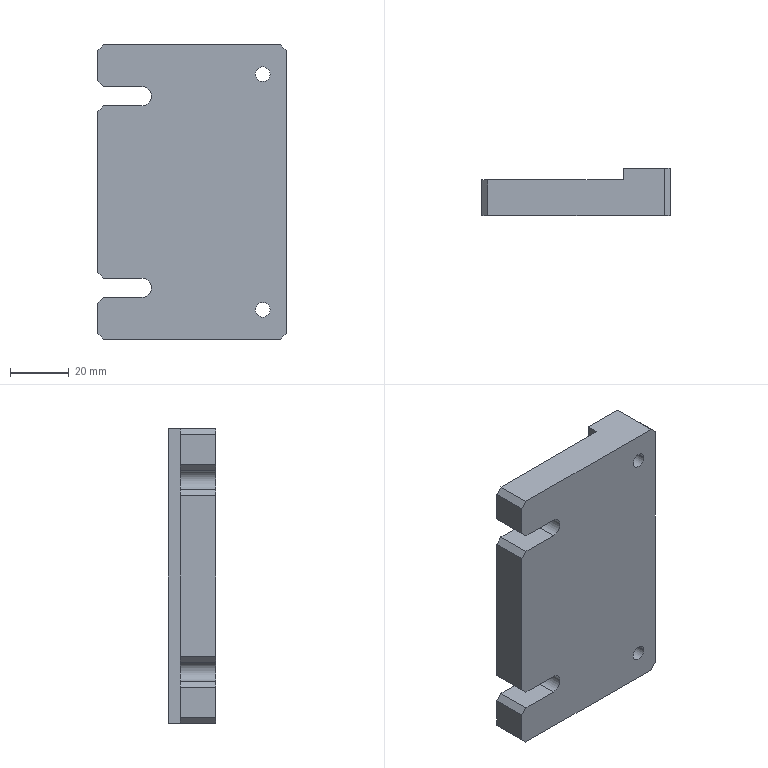Component | SolidWorks | 140507-L01M08U05-2-P03(B)-2 | 1 solid | 28 faces | box 64 x 16 x 100 mm | volume 79625 mm3 | plane 22 | cylinder 6 | commonest cylinder face diameters 5 x4 6.5 x2
build123d program:
from build123d import *

# Parameters (mm, degrees)
SKETCH1_W           = 100
SKETCH1_H           = 64
BOSS_EXTRUDE1_DEPTH = 16
CHAMFER1_SIZE       = 2
M6_TAPPED_HOLE1_D   = 5
CUT_EXTRUDE1_DEPTH  = 62.482
CHAMFER2_SIZE       = 2
SKETCH7_W           = 100
SKETCH7_H           = 48
CUT_EXTRUDE2_DEPTH  = 4


with BuildPart() as part:
    # Sketch1 → Boss-Extrude1 (new body)
    with BuildSketch(Plane(origin=(0, 0, 0), x_dir=(1, 0, 0), z_dir=(0, 1, 0))):
        Rectangle(SKETCH1_W, SKETCH1_H)
    extrude(amount=BOSS_EXTRUDE1_DEPTH)

    # Chamfer1
    chamfer1_edges = [part.edges().sort_by_distance(p)[0] for p in [
        (50, 8, 32),
        (-50, 8, 32),
        (-50, 8, -32),
        (50, 8, -32),
    ]]
    chamfer(chamfer1_edges, length=CHAMFER1_SIZE)

    # M6 Tapped Hole1 (through all)
    with Locations(Plane(origin=(0, 16, 0), x_dir=(1, 0, 0), z_dir=(0, 1, 0))):
        with Locations((-40, 24), (40, 24)):
            Hole(M6_TAPPED_HOLE1_D / 2)

    # Sketch6 → Cut-Extrude1 (cut, through all)
    with BuildSketch(Plane(origin=(0, 16, 0), x_dir=(1, 0, 0), z_dir=(0, 1, 0))):
        with BuildLine():
            Line((-35.75, -32), (-35.75, -17))
            ThreePointArc((-35.75, -17), (-32.5, -13.75), (-29.25, -17))
            Line((-29.25, -17), (-29.25, -32))
            ThreePointArc((-29.25, -32), (-32.5, -35.25), (-35.75, -32))
        make_face()
        with BuildLine():
            Line((35.75, -32), (35.75, -17))
            ThreePointArc((35.75, -17), (32.5, -13.75), (29.25, -17))
            Line((29.25, -17), (29.25, -32))
            ThreePointArc((29.25, -32), (32.5, -35.25), (35.75, -32))
        make_face()
    extrude(amount=-CUT_EXTRUDE1_DEPTH, mode=Mode.SUBTRACT)

    # Chamfer2
    chamfer2_edges = [part.edges().sort_by_distance(p)[0] for p in [
        (-29.25, 8, 32),
        (-35.75, 8, 32),
        (35.75, 8, 32),
        (29.25, 8, 32),
    ]]
    chamfer(chamfer2_edges, length=CHAMFER2_SIZE)

    # Sketch7 → Cut-Extrude2 (cut)
    with BuildSketch(Plane(origin=(0, 16, 0), x_dir=(1, 0, 0), z_dir=(0, 1, 0))):
        with Locations((0, -8)):
            Rectangle(SKETCH7_W, SKETCH7_H)
    extrude(amount=-CUT_EXTRUDE2_DEPTH, mode=Mode.SUBTRACT)


solid = part.part

# Placed as in the assembly
solid = solid.moved(Location((-58.945, -17.656, -21.398), (0, -90, 0)))
STEP:
#1=COLOUR_RGB('',0.7922,0.8196,0.9333);
#2=FILL_AREA_STYLE_COLOUR('',#1);
#3=FILL_AREA_STYLE('',(#2));
#4=SURFACE_STYLE_FILL_AREA(#3);
#5=SURFACE_SIDE_STYLE('',(#4));
#6=SURFACE_STYLE_USAGE(.BOTH.,#5);
#7=PRESENTATION_STYLE_ASSIGNMENT((#6));
#8=CARTESIAN_POINT('',(-1.277,-0.6951,-2.417));
#9=VERTEX_POINT('',#8);
#10=CARTESIAN_POINT('',(-1.474,-0.6951,-2.417));
#11=VERTEX_POINT('',#10);
#12=CARTESIAN_POINT('',(-1.376,-0.6951,-2.417));
#13=DIRECTION('',(0.,1.,0.));
#14=DIRECTION('',(-1.,0.,0.));
#15=AXIS2_PLACEMENT_3D('',#12,#13,#14);
#16=CIRCLE('',#15,0.09843);
#17=EDGE_CURVE('',#9,#11,#16,.T.);
#18=ORIENTED_EDGE('',*,*,#17,.F.);
#19=CARTESIAN_POINT('',(-1.277,-0.0652,-2.417));
#20=VERTEX_POINT('',#19);
#21=CARTESIAN_POINT('',(-1.277,-0.0652,-2.417));
#22=DIRECTION('',(0.,1.,0.));
#23=VECTOR('',#22,39.37);
#24=LINE('',#21,#23);
#25=EDGE_CURVE('',#9,#20,#24,.T.);
#26=ORIENTED_EDGE('',*,*,#25,.T.);
#27=CARTESIAN_POINT('',(-1.474,-0.0652,-2.417));
#28=VERTEX_POINT('',#27);
#29=CARTESIAN_POINT('',(-1.376,-0.0652,-2.417));
#30=DIRECTION('',(0.,1.,0.));
#31=DIRECTION('',(-1.,0.,0.));
#32=AXIS2_PLACEMENT_3D('',#29,#30,#31);
#33=CIRCLE('',#32,0.09843);
#34=EDGE_CURVE('',#20,#28,#33,.T.);
#35=ORIENTED_EDGE('',*,*,#34,.T.);
#36=CARTESIAN_POINT('',(-1.474,-0.0652,-2.417));
#37=DIRECTION('',(0.,1.,0.));
#38=VECTOR('',#37,39.37);
#39=LINE('',#36,#38);
#40=EDGE_CURVE('',#11,#28,#39,.T.);
#41=ORIENTED_EDGE('',*,*,#40,.F.);
#42=EDGE_LOOP('',(#18,#26,#35,#41));
#43=FACE_OUTER_BOUND('',#42,.T.);
#44=CARTESIAN_POINT('',(-1.376,-0.0652,-2.417));
#45=DIRECTION('',(0.,1.,0.));
#46=DIRECTION('',(-1.,0.,0.));
#47=AXIS2_PLACEMENT_3D('',#44,#45,#46);
#48=CYLINDRICAL_SURFACE('',#47,0.09843);
#49=ADVANCED_FACE('',(#43),#48,.F.);
#50=CARTESIAN_POINT('',(-1.277,-0.6951,0.7324));
#51=VERTEX_POINT('',#50);
#52=CARTESIAN_POINT('',(-1.474,-0.6951,0.7324));
#53=VERTEX_POINT('',#52);
#54=CARTESIAN_POINT('',(-1.376,-0.6951,0.7324));
#55=DIRECTION('',(0.,1.,0.));
#56=DIRECTION('',(-1.,0.,0.));
#57=AXIS2_PLACEMENT_3D('',#54,#55,#56);
#58=CIRCLE('',#57,0.09843);
#59=EDGE_CURVE('',#51,#53,#58,.T.);
#60=ORIENTED_EDGE('',*,*,#59,.F.);
#61=CARTESIAN_POINT('',(-1.277,-0.0652,0.7324));
#62=VERTEX_POINT('',#61);
#63=CARTESIAN_POINT('',(-1.277,-0.0652,0.7324));
#64=DIRECTION('',(0.,1.,0.));
#65=VECTOR('',#64,39.37);
#66=LINE('',#63,#65);
#67=EDGE_CURVE('',#51,#62,#66,.T.);
#68=ORIENTED_EDGE('',*,*,#67,.T.);
#69=CARTESIAN_POINT('',(-1.474,-0.0652,0.7324));
#70=VERTEX_POINT('',#69);
#71=CARTESIAN_POINT('',(-1.376,-0.0652,0.7324));
#72=DIRECTION('',(0.,1.,0.));
#73=DIRECTION('',(-1.,0.,0.));
#74=AXIS2_PLACEMENT_3D('',#71,#72,#73);
#75=CIRCLE('',#74,0.09843);
#76=EDGE_CURVE('',#62,#70,#75,.T.);
#77=ORIENTED_EDGE('',*,*,#76,.T.);
#78=CARTESIAN_POINT('',(-1.474,-0.0652,0.7324));
#79=DIRECTION('',(0.,1.,0.));
#80=VECTOR('',#79,39.37);
#81=LINE('',#78,#80);
#82=EDGE_CURVE('',#53,#70,#81,.T.);
#83=ORIENTED_EDGE('',*,*,#82,.F.);
#84=EDGE_LOOP('',(#60,#68,#77,#83));
#85=FACE_OUTER_BOUND('',#84,.T.);
#86=CARTESIAN_POINT('',(-1.376,-0.0652,0.7324));
#87=DIRECTION('',(0.,1.,0.));
#88=DIRECTION('',(-1.,0.,0.));
#89=AXIS2_PLACEMENT_3D('',#86,#87,#88);
#90=CYLINDRICAL_SURFACE('',#89,0.09843);
#91=ADVANCED_FACE('',(#85),#90,.F.);
#92=CARTESIAN_POINT('',(-3.581,-0.2227,-1.915));
#93=VERTEX_POINT('',#92);
#94=CARTESIAN_POINT('',(-3.581,-0.2227,0.2304));
#95=VERTEX_POINT('',#94);
#96=CARTESIAN_POINT('',(-3.581,-0.2227,-2.811));
#97=DIRECTION('',(-0.,-0.,1.));
#98=VECTOR('',#97,39.37);
#99=LINE('',#96,#98);
#100=EDGE_CURVE('',#93,#95,#99,.T.);
#101=ORIENTED_EDGE('',*,*,#100,.F.);
#102=CARTESIAN_POINT('',(-3.581,-0.6951,-1.915));
#103=VERTEX_POINT('',#102);
#104=CARTESIAN_POINT('',(-3.581,-0.0652,-1.915));
#105=DIRECTION('',(-0.,-1.,-0.));
#106=VECTOR('',#105,39.37);
#107=LINE('',#104,#106);
#108=EDGE_CURVE('',#93,#103,#107,.T.);
#109=ORIENTED_EDGE('',*,*,#108,.T.);
#110=CARTESIAN_POINT('',(-3.581,-0.6951,0.2304));
#111=VERTEX_POINT('',#110);
#112=CARTESIAN_POINT('',(-3.581,-0.6951,-2.811));
#113=DIRECTION('',(-0.,-0.,1.));
#114=VECTOR('',#113,39.37);
#115=LINE('',#112,#114);
#116=EDGE_CURVE('',#103,#111,#115,.T.);
#117=ORIENTED_EDGE('',*,*,#116,.T.);
#118=CARTESIAN_POINT('',(-3.581,-0.0652,0.2304));
#119=DIRECTION('',(0.,1.,0.));
#120=VECTOR('',#119,39.37);
#121=LINE('',#118,#120);
#122=EDGE_CURVE('',#111,#95,#121,.T.);
#123=ORIENTED_EDGE('',*,*,#122,.T.);
#124=EDGE_LOOP('',(#101,#109,#117,#123));
#125=FACE_OUTER_BOUND('',#124,.T.);
#126=CARTESIAN_POINT('',(-3.581,-0.0652,-2.811));
#127=DIRECTION('',(1.,-0.,0.));
#128=DIRECTION('',(0.,0.,-1.));
#129=AXIS2_PLACEMENT_3D('',#126,#127,#128);
#130=PLANE('',#129);
#131=ADVANCED_FACE('',(#125),#130,.F.);
#132=CARTESIAN_POINT('',(-3.581,-0.2227,-2.732));
#133=VERTEX_POINT('',#132);
#134=CARTESIAN_POINT('',(-3.581,-0.2227,-2.329));
#135=VERTEX_POINT('',#134);
#136=CARTESIAN_POINT('',(-3.581,-0.2227,-2.811));
#137=DIRECTION('',(-0.,-0.,1.));
#138=VECTOR('',#137,39.37);
#139=LINE('',#136,#138);
#140=EDGE_CURVE('',#133,#135,#139,.T.);
#141=ORIENTED_EDGE('',*,*,#140,.F.);
#142=CARTESIAN_POINT('',(-3.581,-0.6951,-2.732));
#143=VERTEX_POINT('',#142);
#144=CARTESIAN_POINT('',(-3.581,-0.0652,-2.732));
#145=DIRECTION('',(-0.,-1.,-0.));
#146=VECTOR('',#145,39.37);
#147=LINE('',#144,#146);
#148=EDGE_CURVE('',#133,#143,#147,.T.);
#149=ORIENTED_EDGE('',*,*,#148,.T.);
#150=CARTESIAN_POINT('',(-3.581,-0.6951,-2.329));
#151=VERTEX_POINT('',#150);
#152=CARTESIAN_POINT('',(-3.581,-0.6951,-2.811));
#153=DIRECTION('',(-0.,-0.,1.));
#154=VECTOR('',#153,39.37);
#155=LINE('',#152,#154);
#156=EDGE_CURVE('',#143,#151,#155,.T.);
#157=ORIENTED_EDGE('',*,*,#156,.T.);
#158=CARTESIAN_POINT('',(-3.581,-0.0652,-2.329));
#159=DIRECTION('',(0.,1.,0.));
#160=VECTOR('',#159,39.37);
#161=LINE('',#158,#160);
#162=EDGE_CURVE('',#151,#135,#161,.T.);
#163=ORIENTED_EDGE('',*,*,#162,.T.);
#164=EDGE_LOOP('',(#141,#149,#157,#163));
#165=FACE_OUTER_BOUND('',#164,.T.);
#166=CARTESIAN_POINT('',(-3.581,-0.0652,-2.811));
#167=DIRECTION('',(1.,-0.,0.));
#168=DIRECTION('',(0.,0.,-1.));
#169=AXIS2_PLACEMENT_3D('',#166,#167,#168);
#170=PLANE('',#169);
#171=ADVANCED_FACE('',(#165),#170,.F.);
#172=CARTESIAN_POINT('',(-3.581,-0.2227,0.6438));
#173=VERTEX_POINT('',#172);
#174=CARTESIAN_POINT('',(-3.581,-0.2227,1.047));
#175=VERTEX_POINT('',#174);
#176=CARTESIAN_POINT('',(-3.581,-0.2227,-2.811));
#177=DIRECTION('',(-0.,-0.,1.));
#178=VECTOR('',#177,39.37);
#179=LINE('',#176,#178);
#180=EDGE_CURVE('',#173,#175,#179,.T.);
#181=ORIENTED_EDGE('',*,*,#180,.F.);
#182=CARTESIAN_POINT('',(-3.581,-0.6951,0.6438));
#183=VERTEX_POINT('',#182);
#184=CARTESIAN_POINT('',(-3.581,-0.0652,0.6438));
#185=DIRECTION('',(-0.,-1.,-0.));
#186=VECTOR('',#185,39.37);
#187=LINE('',#184,#186);
#188=EDGE_CURVE('',#173,#183,#187,.T.);
#189=ORIENTED_EDGE('',*,*,#188,.T.);
#190=CARTESIAN_POINT('',(-3.581,-0.6951,1.047));
#191=VERTEX_POINT('',#190);
#192=CARTESIAN_POINT('',(-3.581,-0.6951,-2.811));
#193=DIRECTION('',(-0.,-0.,1.));
#194=VECTOR('',#193,39.37);
#195=LINE('',#192,#194);
#196=EDGE_CURVE('',#183,#191,#195,.T.);
#197=ORIENTED_EDGE('',*,*,#196,.T.);
#198=CARTESIAN_POINT('',(-3.581,-0.0652,1.047));
#199=DIRECTION('',(0.,1.,0.));
#200=VECTOR('',#199,39.37);
#201=LINE('',#198,#200);
#202=EDGE_CURVE('',#191,#175,#201,.T.);
#203=ORIENTED_EDGE('',*,*,#202,.T.);
#204=EDGE_LOOP('',(#181,#189,#197,#203));
#205=FACE_OUTER_BOUND('',#204,.T.);
#206=CARTESIAN_POINT('',(-3.581,-0.0652,-2.811));
#207=DIRECTION('',(1.,-0.,0.));
#208=DIRECTION('',(0.,0.,-1.));
#209=AXIS2_PLACEMENT_3D('',#206,#207,#208);
#210=PLANE('',#209);
#211=ADVANCED_FACE('',(#205),#210,.F.);
#212=CARTESIAN_POINT('',(-3.502,-0.2227,1.126));
#213=VERTEX_POINT('',#212);
#214=CARTESIAN_POINT('',(-3.502,-0.6951,1.126));
#215=VERTEX_POINT('',#214);
#216=CARTESIAN_POINT('',(-3.502,-0.0652,1.126));
#217=DIRECTION('',(-0.,-1.,-0.));
#218=VECTOR('',#217,39.37);
#219=LINE('',#216,#218);
#220=EDGE_CURVE('',#213,#215,#219,.T.);
#221=ORIENTED_EDGE('',*,*,#220,.F.);
#222=CARTESIAN_POINT('',(-3.502,-0.2227,1.126));
#223=DIRECTION('',(-0.7071,0.,-0.7071));
#224=VECTOR('',#223,39.37);
#225=LINE('',#222,#224);
#226=EDGE_CURVE('',#213,#175,#225,.T.);
#227=ORIENTED_EDGE('',*,*,#226,.T.);
#228=ORIENTED_EDGE('',*,*,#202,.F.);
#229=CARTESIAN_POINT('',(-3.502,-0.6951,1.126));
#230=DIRECTION('',(-0.7071,0.,-0.7071));
#231=VECTOR('',#230,39.37);
#232=LINE('',#229,#231);
#233=EDGE_CURVE('',#215,#191,#232,.T.);
#234=ORIENTED_EDGE('',*,*,#233,.F.);
#235=EDGE_LOOP('',(#221,#227,#228,#234));
#236=FACE_OUTER_BOUND('',#235,.T.);
#237=CARTESIAN_POINT('',(-3.502,-0.0652,1.126));
#238=DIRECTION('',(0.7071,-0.,-0.7071));
#239=DIRECTION('',(-0.,-1.,-0.));
#240=AXIS2_PLACEMENT_3D('',#237,#238,#239);
#241=PLANE('',#240);
#242=ADVANCED_FACE('',(#236),#241,.F.);
#243=ORIENTED_EDGE('',*,*,#148,.F.);
#244=CARTESIAN_POINT('',(-3.502,-0.2227,-2.811));
#245=VERTEX_POINT('',#244);
#246=CARTESIAN_POINT('',(-3.581,-0.2227,-2.732));
#247=DIRECTION('',(0.7071,-0.,-0.7071));
#248=VECTOR('',#247,39.37);
#249=LINE('',#246,#248);
#250=EDGE_CURVE('',#133,#245,#249,.T.);
#251=ORIENTED_EDGE('',*,*,#250,.T.);
#252=CARTESIAN_POINT('',(-3.502,-0.6951,-2.811));
#253=VERTEX_POINT('',#252);
#254=CARTESIAN_POINT('',(-3.502,-0.0652,-2.811));
#255=DIRECTION('',(0.,1.,0.));
#256=VECTOR('',#255,39.37);
#257=LINE('',#254,#256);
#258=EDGE_CURVE('',#253,#245,#257,.T.);
#259=ORIENTED_EDGE('',*,*,#258,.F.);
#260=CARTESIAN_POINT('',(-3.581,-0.6951,-2.732));
#261=DIRECTION('',(0.7071,-0.,-0.7071));
#262=VECTOR('',#261,39.37);
#263=LINE('',#260,#262);
#264=EDGE_CURVE('',#143,#253,#263,.T.);
#265=ORIENTED_EDGE('',*,*,#264,.F.);
#266=EDGE_LOOP('',(#243,#251,#259,#265));
#267=FACE_OUTER_BOUND('',#266,.T.);
#268=CARTESIAN_POINT('',(-3.581,-0.0652,-2.732));
#269=DIRECTION('',(0.7071,-0.,0.7071));
#270=DIRECTION('',(-0.,-1.,-0.));
#271=AXIS2_PLACEMENT_3D('',#268,#269,#270);
#272=PLANE('',#271);
#273=ADVANCED_FACE('',(#267),#272,.F.);
#274=CARTESIAN_POINT('',(-3.502,-0.2227,-2.25));
#275=VERTEX_POINT('',#274);
#276=CARTESIAN_POINT('',(-2.99,-0.2227,-2.25));
#277=VERTEX_POINT('',#276);
#278=CARTESIAN_POINT('',(-3.581,-0.2227,-2.25));
#279=DIRECTION('',(1.,-0.,0.));
#280=VECTOR('',#279,39.37);
#281=LINE('',#278,#280);
#282=EDGE_CURVE('',#275,#277,#281,.T.);
#283=ORIENTED_EDGE('',*,*,#282,.F.);
#284=CARTESIAN_POINT('',(-3.502,-0.6951,-2.25));
#285=VERTEX_POINT('',#284);
#286=CARTESIAN_POINT('',(-3.502,-0.6951,-2.25));
#287=DIRECTION('',(-0.,-1.,-0.));
#288=VECTOR('',#287,39.37);
#289=LINE('',#286,#288);
#290=EDGE_CURVE('',#275,#285,#289,.T.);
#291=ORIENTED_EDGE('',*,*,#290,.T.);
#292=CARTESIAN_POINT('',(-2.99,-0.6951,-2.25));
#293=VERTEX_POINT('',#292);
#294=CARTESIAN_POINT('',(-3.581,-0.6951,-2.25));
#295=DIRECTION('',(-1.,0.,-0.));
#296=VECTOR('',#295,39.37);
#297=LINE('',#294,#296);
#298=EDGE_CURVE('',#293,#285,#297,.T.);
#299=ORIENTED_EDGE('',*,*,#298,.F.);
#300=CARTESIAN_POINT('',(-2.99,-0.6951,-2.25));
#301=DIRECTION('',(0.,1.,0.));
#302=VECTOR('',#301,39.37);
#303=LINE('',#300,#302);
#304=EDGE_CURVE('',#293,#277,#303,.T.);
#305=ORIENTED_EDGE('',*,*,#304,.T.);
#306=EDGE_LOOP('',(#283,#291,#299,#305));
#307=FACE_OUTER_BOUND('',#306,.T.);
#308=CARTESIAN_POINT('',(-3.581,-0.6951,-2.25));
#309=DIRECTION('',(0.,0.,-1.));
#310=DIRECTION('',(-1.,0.,-0.));
#311=AXIS2_PLACEMENT_3D('',#308,#309,#310);
#312=PLANE('',#311);
#313=ADVANCED_FACE('',(#307),#312,.F.);
#314=CARTESIAN_POINT('',(-2.99,-0.2227,-1.994));
#315=VERTEX_POINT('',#314);
#316=CARTESIAN_POINT('',(-2.99,-0.2227,-2.122));
#317=DIRECTION('',(-0.,-1.,-0.));
#318=DIRECTION('',(-1.,0.,0.));
#319=AXIS2_PLACEMENT_3D('',#316,#317,#318);
#320=CIRCLE('',#319,0.128);
#321=EDGE_CURVE('',#277,#315,#320,.T.);
#322=ORIENTED_EDGE('',*,*,#321,.F.);
#323=ORIENTED_EDGE('',*,*,#304,.F.);
#324=CARTESIAN_POINT('',(-2.99,-0.6951,-1.994));
#325=VERTEX_POINT('',#324);
#326=CARTESIAN_POINT('',(-2.99,-0.6951,-2.122));
#327=DIRECTION('',(0.,1.,0.));
#328=DIRECTION('',(-1.,0.,0.));
#329=AXIS2_PLACEMENT_3D('',#326,#327,#328);
#330=CIRCLE('',#329,0.128);
#331=EDGE_CURVE('',#325,#293,#330,.T.);
#332=ORIENTED_EDGE('',*,*,#331,.F.);
#333=CARTESIAN_POINT('',(-2.99,-0.6951,-1.994));
#334=DIRECTION('',(0.,1.,0.));
#335=VECTOR('',#334,39.37);
#336=LINE('',#333,#335);
#337=EDGE_CURVE('',#325,#315,#336,.T.);
#338=ORIENTED_EDGE('',*,*,#337,.T.);
#339=EDGE_LOOP('',(#322,#323,#332,#338));
#340=FACE_OUTER_BOUND('',#339,.T.);
#341=CARTESIAN_POINT('',(-2.99,-0.6951,-2.122));
#342=DIRECTION('',(0.,1.,0.));
#343=DIRECTION('',(-1.,0.,0.));
#344=AXIS2_PLACEMENT_3D('',#341,#342,#343);
#345=CYLINDRICAL_SURFACE('',#344,0.128);
#346=ADVANCED_FACE('',(#340),#345,.F.);
#347=CARTESIAN_POINT('',(-3.502,-0.2227,-1.994));
#348=VERTEX_POINT('',#347);
#349=CARTESIAN_POINT('',(-3.581,-0.2227,-1.994));
#350=DIRECTION('',(-1.,0.,-0.));
#351=VECTOR('',#350,39.37);
#352=LINE('',#349,#351);
#353=EDGE_CURVE('',#315,#348,#352,.T.);
#354=ORIENTED_EDGE('',*,*,#353,.F.);
#355=ORIENTED_EDGE('',*,*,#337,.F.);
#356=CARTESIAN_POINT('',(-3.502,-0.6951,-1.994));
#357=VERTEX_POINT('',#356);
#358=CARTESIAN_POINT('',(-3.581,-0.6951,-1.994));
#359=DIRECTION('',(1.,-0.,0.));
#360=VECTOR('',#359,39.37);
#361=LINE('',#358,#360);
#362=EDGE_CURVE('',#357,#325,#361,.T.);
#363=ORIENTED_EDGE('',*,*,#362,.F.);
#364=CARTESIAN_POINT('',(-3.502,-0.6951,-1.994));
#365=DIRECTION('',(0.,1.,0.));
#366=VECTOR('',#365,39.37);
#367=LINE('',#364,#366);
#368=EDGE_CURVE('',#357,#348,#367,.T.);
#369=ORIENTED_EDGE('',*,*,#368,.T.);
#370=EDGE_LOOP('',(#354,#355,#363,#369));
#371=FACE_OUTER_BOUND('',#370,.T.);
#372=CARTESIAN_POINT('',(-3.581,-0.6951,-1.994));
#373=DIRECTION('',(-0.,-0.,1.));
#374=DIRECTION('',(1.,-0.,0.));
#375=AXIS2_PLACEMENT_3D('',#372,#373,#374);
#376=PLANE('',#375);
#377=ADVANCED_FACE('',(#371),#376,.F.);
#378=CARTESIAN_POINT('',(-3.502,-0.2227,0.3091));
#379=VERTEX_POINT('',#378);
#380=CARTESIAN_POINT('',(-2.99,-0.2227,0.3091));
#381=VERTEX_POINT('',#380);
#382=CARTESIAN_POINT('',(-3.581,-0.2227,0.3091));
#383=DIRECTION('',(1.,-0.,0.));
#384=VECTOR('',#383,39.37);
#385=LINE('',#382,#384);
#386=EDGE_CURVE('',#379,#381,#385,.T.);
#387=ORIENTED_EDGE('',*,*,#386,.F.);
#388=CARTESIAN_POINT('',(-3.502,-0.6951,0.3091));
#389=VERTEX_POINT('',#388);
#390=CARTESIAN_POINT('',(-3.502,-0.6951,0.3091));
#391=DIRECTION('',(-0.,-1.,-0.));
#392=VECTOR('',#391,39.37);
#393=LINE('',#390,#392);
#394=EDGE_CURVE('',#379,#389,#393,.T.);
#395=ORIENTED_EDGE('',*,*,#394,.T.);
#396=CARTESIAN_POINT('',(-2.99,-0.6951,0.3091));
#397=VERTEX_POINT('',#396);
#398=CARTESIAN_POINT('',(-3.581,-0.6951,0.3091));
#399=DIRECTION('',(-1.,0.,-0.));
#400=VECTOR('',#399,39.37);
#401=LINE('',#398,#400);
#402=EDGE_CURVE('',#397,#389,#401,.T.);
#403=ORIENTED_EDGE('',*,*,#402,.F.);
#404=CARTESIAN_POINT('',(-2.99,-0.6951,0.3091));
#405=DIRECTION('',(0.,1.,0.));
#406=VECTOR('',#405,39.37);
#407=LINE('',#404,#406);
#408=EDGE_CURVE('',#397,#381,#407,.T.);
#409=ORIENTED_EDGE('',*,*,#408,.T.);
#410=EDGE_LOOP('',(#387,#395,#403,#409));
#411=FACE_OUTER_BOUND('',#410,.T.);
#412=CARTESIAN_POINT('',(-3.581,-0.6951,0.3091));
#413=DIRECTION('',(0.,0.,-1.));
#414=DIRECTION('',(-1.,0.,-0.));
#415=AXIS2_PLACEMENT_3D('',#412,#413,#414);
#416=PLANE('',#415);
#417=ADVANCED_FACE('',(#411),#416,.F.);
#418=CARTESIAN_POINT('',(-2.99,-0.2227,0.565));
#419=VERTEX_POINT('',#418);
#420=CARTESIAN_POINT('',(-2.99,-0.2227,0.4371));
#421=DIRECTION('',(-0.,-1.,-0.));
#422=DIRECTION('',(-1.,0.,0.));
#423=AXIS2_PLACEMENT_3D('',#420,#421,#422);
#424=CIRCLE('',#423,0.128);
#425=EDGE_CURVE('',#381,#419,#424,.T.);
#426=ORIENTED_EDGE('',*,*,#425,.F.);
#427=ORIENTED_EDGE('',*,*,#408,.F.);
#428=CARTESIAN_POINT('',(-2.99,-0.6951,0.565));
#429=VERTEX_POINT('',#428);
#430=CARTESIAN_POINT('',(-2.99,-0.6951,0.4371));
#431=DIRECTION('',(0.,1.,0.));
#432=DIRECTION('',(1.,0.,0.));
#433=AXIS2_PLACEMENT_3D('',#430,#431,#432);
#434=CIRCLE('',#433,0.128);
#435=EDGE_CURVE('',#429,#397,#434,.T.);
#436=ORIENTED_EDGE('',*,*,#435,.F.);
#437=CARTESIAN_POINT('',(-2.99,-0.6951,0.565));
#438=DIRECTION('',(0.,1.,0.));
#439=VECTOR('',#438,39.37);
#440=LINE('',#437,#439);
#441=EDGE_CURVE('',#429,#419,#440,.T.);
#442=ORIENTED_EDGE('',*,*,#441,.T.);
#443=EDGE_LOOP('',(#426,#427,#436,#442));
#444=FACE_OUTER_BOUND('',#443,.T.);
#445=CARTESIAN_POINT('',(-2.99,-0.6951,0.4371));
#446=DIRECTION('',(0.,1.,0.));
#447=DIRECTION('',(-1.,0.,0.));
#448=AXIS2_PLACEMENT_3D('',#445,#446,#447);
#449=CYLINDRICAL_SURFACE('',#448,0.128);
#450=ADVANCED_FACE('',(#444),#449,.F.);
#451=CARTESIAN_POINT('',(-3.502,-0.2227,0.565));
#452=VERTEX_POINT('',#451);
#453=CARTESIAN_POINT('',(-3.581,-0.2227,0.565));
#454=DIRECTION('',(-1.,0.,-0.));
#455=VECTOR('',#454,39.37);
#456=LINE('',#453,#455);
#457=EDGE_CURVE('',#419,#452,#456,.T.);
#458=ORIENTED_EDGE('',*,*,#457,.F.);
#459=ORIENTED_EDGE('',*,*,#441,.F.);
#460=CARTESIAN_POINT('',(-3.502,-0.6951,0.565));
#461=VERTEX_POINT('',#460);
#462=CARTESIAN_POINT('',(-3.581,-0.6951,0.565));
#463=DIRECTION('',(1.,-0.,0.));
#464=VECTOR('',#463,39.37);
#465=LINE('',#462,#464);
#466=EDGE_CURVE('',#461,#429,#465,.T.);
#467=ORIENTED_EDGE('',*,*,#466,.F.);
#468=CARTESIAN_POINT('',(-3.502,-0.6951,0.565));
#469=DIRECTION('',(0.,1.,0.));
#470=VECTOR('',#469,39.37);
#471=LINE('',#468,#470);
#472=EDGE_CURVE('',#461,#452,#471,.T.);
#473=ORIENTED_EDGE('',*,*,#472,.T.);
#474=EDGE_LOOP('',(#458,#459,#467,#473));
#475=FACE_OUTER_BOUND('',#474,.T.);
#476=CARTESIAN_POINT('',(-3.581,-0.6951,0.565));
#477=DIRECTION('',(-0.,-0.,1.));
#478=DIRECTION('',(1.,-0.,0.));
#479=AXIS2_PLACEMENT_3D('',#476,#477,#478);
#480=PLANE('',#479);
#481=ADVANCED_FACE('',(#475),#480,.F.);
#482=ORIENTED_EDGE('',*,*,#188,.F.);
#483=CARTESIAN_POINT('',(-3.502,-0.2227,0.565));
#484=DIRECTION('',(0.7071,-0.,-0.7071));
#485=VECTOR('',#484,39.37);
#486=LINE('',#483,#485);
#487=EDGE_CURVE('',#173,#452,#486,.T.);
#488=ORIENTED_EDGE('',*,*,#487,.T.);
#489=ORIENTED_EDGE('',*,*,#472,.F.);
#490=CARTESIAN_POINT('',(-3.502,-0.6951,0.565));
#491=DIRECTION('',(0.7071,-0.,-0.7071));
#492=VECTOR('',#491,39.37);
#493=LINE('',#490,#492);
#494=EDGE_CURVE('',#183,#461,#493,.T.);
#495=ORIENTED_EDGE('',*,*,#494,.F.);
#496=EDGE_LOOP('',(#482,#488,#489,#495));
#497=FACE_OUTER_BOUND('',#496,.T.);
#498=CARTESIAN_POINT('',(-3.502,-0.6951,0.565));
#499=DIRECTION('',(0.7071,-0.,0.7071));
#500=DIRECTION('',(0.,1.,0.));
#501=AXIS2_PLACEMENT_3D('',#498,#499,#500);
#502=PLANE('',#501);
#503=ADVANCED_FACE('',(#497),#502,.F.);
#504=ORIENTED_EDGE('',*,*,#394,.F.);
#505=CARTESIAN_POINT('',(-3.581,-0.2227,0.2304));
#506=DIRECTION('',(-0.7071,0.,-0.7071));
#507=VECTOR('',#506,39.37);
#508=LINE('',#505,#507);
#509=EDGE_CURVE('',#379,#95,#508,.T.);
#510=ORIENTED_EDGE('',*,*,#509,.T.);
#511=ORIENTED_EDGE('',*,*,#122,.F.);
#512=CARTESIAN_POINT('',(-3.581,-0.6951,0.2304));
#513=DIRECTION('',(-0.7071,0.,-0.7071));
#514=VECTOR('',#513,39.37);
#515=LINE('',#512,#514);
#516=EDGE_CURVE('',#389,#111,#515,.T.);
#517=ORIENTED_EDGE('',*,*,#516,.F.);
#518=EDGE_LOOP('',(#504,#510,#511,#517));
#519=FACE_OUTER_BOUND('',#518,.T.);
#520=CARTESIAN_POINT('',(-3.581,-0.0652,0.2304));
#521=DIRECTION('',(0.7071,-0.,-0.7071));
#522=DIRECTION('',(0.,1.,0.));
#523=AXIS2_PLACEMENT_3D('',#520,#521,#522);
#524=PLANE('',#523);
#525=ADVANCED_FACE('',(#519),#524,.F.);
#526=ORIENTED_EDGE('',*,*,#108,.F.);
#527=CARTESIAN_POINT('',(-3.502,-0.2227,-1.994));
#528=DIRECTION('',(0.7071,-0.,-0.7071));
#529=VECTOR('',#528,39.37);
#530=LINE('',#527,#529);
#531=EDGE_CURVE('',#93,#348,#530,.T.);
#532=ORIENTED_EDGE('',*,*,#531,.T.);
#533=ORIENTED_EDGE('',*,*,#368,.F.);
#534=CARTESIAN_POINT('',(-3.502,-0.6951,-1.994));
#535=DIRECTION('',(0.7071,-0.,-0.7071));
#536=VECTOR('',#535,39.37);
#537=LINE('',#534,#536);
#538=EDGE_CURVE('',#103,#357,#537,.T.);
#539=ORIENTED_EDGE('',*,*,#538,.F.);
#540=EDGE_LOOP('',(#526,#532,#533,#539));
#541=FACE_OUTER_BOUND('',#540,.T.);
#542=CARTESIAN_POINT('',(-3.502,-0.6951,-1.994));
#543=DIRECTION('',(0.7071,-0.,0.7071));
#544=DIRECTION('',(0.,1.,0.));
#545=AXIS2_PLACEMENT_3D('',#542,#543,#544);
#546=PLANE('',#545);
#547=ADVANCED_FACE('',(#541),#546,.F.);
#548=ORIENTED_EDGE('',*,*,#290,.F.);
#549=CARTESIAN_POINT('',(-3.581,-0.2227,-2.329));
#550=DIRECTION('',(-0.7071,0.,-0.7071));
#551=VECTOR('',#550,39.37);
#552=LINE('',#549,#551);
#553=EDGE_CURVE('',#275,#135,#552,.T.);
#554=ORIENTED_EDGE('',*,*,#553,.T.);
#555=ORIENTED_EDGE('',*,*,#162,.F.);
#556=CARTESIAN_POINT('',(-3.581,-0.6951,-2.329));
#557=DIRECTION('',(-0.7071,0.,-0.7071));
#558=VECTOR('',#557,39.37);
#559=LINE('',#556,#558);
#560=EDGE_CURVE('',#285,#151,#559,.T.);
#561=ORIENTED_EDGE('',*,*,#560,.F.);
#562=EDGE_LOOP('',(#548,#554,#555,#561));
#563=FACE_OUTER_BOUND('',#562,.T.);
#564=CARTESIAN_POINT('',(-3.581,-0.0652,-2.329));
#565=DIRECTION('',(0.7071,-0.,-0.7071));
#566=DIRECTION('',(0.,1.,0.));
#567=AXIS2_PLACEMENT_3D('',#564,#565,#566);
#568=PLANE('',#567);
#569=ADVANCED_FACE('',(#563),#568,.F.);
#570=CARTESIAN_POINT('',(-1.691,-0.0652,1.126));
#571=VERTEX_POINT('',#570);
#572=CARTESIAN_POINT('',(-1.14,-0.0652,1.126));
#573=VERTEX_POINT('',#572);
#574=CARTESIAN_POINT('',(-1.061,-0.0652,1.126));
#575=DIRECTION('',(1.,-0.,-0.));
#576=VECTOR('',#575,39.37);
#577=LINE('',#574,#576);
#578=EDGE_CURVE('',#571,#573,#577,.T.);
#579=ORIENTED_EDGE('',*,*,#578,.F.);
#580=CARTESIAN_POINT('',(-1.691,-0.2227,1.126));
#581=VERTEX_POINT('',#580);
#582=CARTESIAN_POINT('',(-1.691,-0.2227,1.126));
#583=DIRECTION('',(0.,1.,0.));
#584=VECTOR('',#583,39.37);
#585=LINE('',#582,#584);
#586=EDGE_CURVE('',#581,#571,#585,.T.);
#587=ORIENTED_EDGE('',*,*,#586,.F.);
#588=CARTESIAN_POINT('',(-1.691,-0.2227,1.126));
#589=DIRECTION('',(1.,-0.,0.));
#590=VECTOR('',#589,39.37);
#591=LINE('',#588,#590);
#592=EDGE_CURVE('',#213,#581,#591,.T.);
#593=ORIENTED_EDGE('',*,*,#592,.F.);
#594=ORIENTED_EDGE('',*,*,#220,.T.);
#595=CARTESIAN_POINT('',(-1.14,-0.6951,1.126));
#596=VERTEX_POINT('',#595);
#597=CARTESIAN_POINT('',(-1.061,-0.6951,1.126));
#598=DIRECTION('',(1.,-0.,-0.));
#599=VECTOR('',#598,39.37);
#600=LINE('',#597,#599);
#601=EDGE_CURVE('',#215,#596,#600,.T.);
#602=ORIENTED_EDGE('',*,*,#601,.T.);
#603=CARTESIAN_POINT('',(-1.14,-0.0652,1.126));
#604=DIRECTION('',(0.,1.,0.));
#605=VECTOR('',#604,39.37);
#606=LINE('',#603,#605);
#607=EDGE_CURVE('',#596,#573,#606,.T.);
#608=ORIENTED_EDGE('',*,*,#607,.T.);
#609=EDGE_LOOP('',(#579,#587,#593,#594,#602,#608));
#610=FACE_OUTER_BOUND('',#609,.T.);
#611=CARTESIAN_POINT('',(-1.061,-0.0652,1.126));
#612=DIRECTION('',(-0.,0.,-1.));
#613=DIRECTION('',(-1.,0.,0.));
#614=AXIS2_PLACEMENT_3D('',#611,#612,#613);
#615=PLANE('',#614);
#616=ADVANCED_FACE('',(#610),#615,.F.);
#617=CARTESIAN_POINT('',(-1.061,-0.0652,1.047));
#618=VERTEX_POINT('',#617);
#619=CARTESIAN_POINT('',(-1.061,-0.0652,-2.732));
#620=VERTEX_POINT('',#619);
#621=CARTESIAN_POINT('',(-1.061,-0.0652,-2.811));
#622=DIRECTION('',(0.,0.,-1.));
#623=VECTOR('',#622,39.37);
#624=LINE('',#621,#623);
#625=EDGE_CURVE('',#618,#620,#624,.T.);
#626=ORIENTED_EDGE('',*,*,#625,.F.);
#627=CARTESIAN_POINT('',(-1.061,-0.6951,1.047));
#628=VERTEX_POINT('',#627);
#629=CARTESIAN_POINT('',(-1.061,-0.0652,1.047));
#630=DIRECTION('',(-0.,-1.,-0.));
#631=VECTOR('',#630,39.37);
#632=LINE('',#629,#631);
#633=EDGE_CURVE('',#618,#628,#632,.T.);
#634=ORIENTED_EDGE('',*,*,#633,.T.);
#635=CARTESIAN_POINT('',(-1.061,-0.6951,-2.732));
#636=VERTEX_POINT('',#635);
#637=CARTESIAN_POINT('',(-1.061,-0.6951,-2.811));
#638=DIRECTION('',(0.,0.,-1.));
#639=VECTOR('',#638,39.37);
#640=LINE('',#637,#639);
#641=EDGE_CURVE('',#628,#636,#640,.T.);
#642=ORIENTED_EDGE('',*,*,#641,.T.);
#643=CARTESIAN_POINT('',(-1.061,-0.0652,-2.732));
#644=DIRECTION('',(0.,1.,0.));
#645=VECTOR('',#644,39.37);
#646=LINE('',#643,#645);
#647=EDGE_CURVE('',#636,#620,#646,.T.);
#648=ORIENTED_EDGE('',*,*,#647,.T.);
#649=EDGE_LOOP('',(#626,#634,#642,#648));
#650=FACE_OUTER_BOUND('',#649,.T.);
#651=CARTESIAN_POINT('',(-1.061,-0.0652,-2.811));
#652=DIRECTION('',(-1.,0.,-0.));
#653=DIRECTION('',(-0.,-0.,1.));
#654=AXIS2_PLACEMENT_3D('',#651,#652,#653);
#655=PLANE('',#654);
#656=ADVANCED_FACE('',(#650),#655,.F.);
#657=CARTESIAN_POINT('',(-1.691,-0.2227,-2.811));
#658=VERTEX_POINT('',#657);
#659=CARTESIAN_POINT('',(-1.691,-0.2227,-2.811));
#660=DIRECTION('',(-1.,0.,-0.));
#661=VECTOR('',#660,39.37);
#662=LINE('',#659,#661);
#663=EDGE_CURVE('',#658,#245,#662,.T.);
#664=ORIENTED_EDGE('',*,*,#663,.F.);
#665=CARTESIAN_POINT('',(-1.691,-0.0652,-2.811));
#666=VERTEX_POINT('',#665);
#667=CARTESIAN_POINT('',(-1.691,-0.2227,-2.811));
#668=DIRECTION('',(0.,1.,0.));
#669=VECTOR('',#668,39.37);
#670=LINE('',#667,#669);
#671=EDGE_CURVE('',#658,#666,#670,.T.);
#672=ORIENTED_EDGE('',*,*,#671,.T.);
#673=CARTESIAN_POINT('',(-1.14,-0.0652,-2.811));
#674=VERTEX_POINT('',#673);
#675=CARTESIAN_POINT('',(-1.061,-0.0652,-2.811));
#676=DIRECTION('',(-1.,0.,0.));
#677=VECTOR('',#676,39.37);
#678=LINE('',#675,#677);
#679=EDGE_CURVE('',#674,#666,#678,.T.);
#680=ORIENTED_EDGE('',*,*,#679,.F.);
#681=CARTESIAN_POINT('',(-1.14,-0.6951,-2.811));
#682=VERTEX_POINT('',#681);
#683=CARTESIAN_POINT('',(-1.14,-0.0652,-2.811));
#684=DIRECTION('',(-0.,-1.,-0.));
#685=VECTOR('',#684,39.37);
#686=LINE('',#683,#685);
#687=EDGE_CURVE('',#674,#682,#686,.T.);
#688=ORIENTED_EDGE('',*,*,#687,.T.);
#689=CARTESIAN_POINT('',(-1.061,-0.6951,-2.811));
#690=DIRECTION('',(-1.,0.,0.));
#691=VECTOR('',#690,39.37);
#692=LINE('',#689,#691);
#693=EDGE_CURVE('',#682,#253,#692,.T.);
#694=ORIENTED_EDGE('',*,*,#693,.T.);
#695=ORIENTED_EDGE('',*,*,#258,.T.);
#696=EDGE_LOOP('',(#664,#672,#680,#688,#694,#695));
#697=FACE_OUTER_BOUND('',#696,.T.);
#698=CARTESIAN_POINT('',(-1.061,-0.0652,-2.811));
#699=DIRECTION('',(0.,-0.,1.));
#700=DIRECTION('',(1.,-0.,-0.));
#701=AXIS2_PLACEMENT_3D('',#698,#699,#700);
#702=PLANE('',#701);
#703=ADVANCED_FACE('',(#697),#702,.F.);
#704=CARTESIAN_POINT('',(-1.691,-0.0652,-2.811));
#705=DIRECTION('',(0.,0.,-1.));
#706=VECTOR('',#705,39.37);
#707=LINE('',#704,#706);
#708=EDGE_CURVE('',#571,#666,#707,.T.);
#709=ORIENTED_EDGE('',*,*,#708,.F.);
#710=ORIENTED_EDGE('',*,*,#578,.T.);
#711=CARTESIAN_POINT('',(-0.7459,-0.0652,0.7324));
#712=DIRECTION('',(0.7071,-0.,-0.7071));
#713=VECTOR('',#712,39.37);
#714=LINE('',#711,#713);
#715=EDGE_CURVE('',#573,#618,#714,.T.);
#716=ORIENTED_EDGE('',*,*,#715,.T.);
#717=ORIENTED_EDGE('',*,*,#625,.T.);
#718=CARTESIAN_POINT('',(-0.7459,-0.0652,-2.417));
#719=DIRECTION('',(-0.7071,0.,-0.7071));
#720=VECTOR('',#719,39.37);
#721=LINE('',#718,#720);
#722=EDGE_CURVE('',#620,#674,#721,.T.);
#723=ORIENTED_EDGE('',*,*,#722,.T.);
#724=ORIENTED_EDGE('',*,*,#679,.T.);
#725=EDGE_LOOP('',(#709,#710,#716,#717,#723,#724));
#726=FACE_OUTER_BOUND('',#725,.T.);
#727=CARTESIAN_POINT('',(-1.376,-0.0652,-2.417));
#728=DIRECTION('',(0.,1.,0.));
#729=DIRECTION('',(-1.,0.,0.));
#730=AXIS2_PLACEMENT_3D('',#727,#728,#729);
#731=CIRCLE('',#730,0.09843);
#732=EDGE_CURVE('',#28,#20,#731,.T.);
#733=ORIENTED_EDGE('',*,*,#732,.F.);
#734=ORIENTED_EDGE('',*,*,#34,.F.);
#735=EDGE_LOOP('',(#733,#734));
#736=FACE_BOUND('',#735,.T.);
#737=CARTESIAN_POINT('',(-1.376,-0.0652,0.7324));
#738=DIRECTION('',(0.,1.,0.));
#739=DIRECTION('',(-1.,0.,0.));
#740=AXIS2_PLACEMENT_3D('',#737,#738,#739);
#741=CIRCLE('',#740,0.09843);
#742=EDGE_CURVE('',#70,#62,#741,.T.);
#743=ORIENTED_EDGE('',*,*,#742,.F.);
#744=ORIENTED_EDGE('',*,*,#76,.F.);
#745=EDGE_LOOP('',(#743,#744));
#746=FACE_BOUND('',#745,.T.);
#747=CARTESIAN_POINT('',(-2.321,-0.0652,-0.8424));
#748=DIRECTION('',(0.,1.,0.));
#749=DIRECTION('',(-1.,0.,-0.));
#750=AXIS2_PLACEMENT_3D('',#747,#748,#749);
#751=PLANE('',#750);
#752=ADVANCED_FACE('',(#726,#736,#746),#751,.T.);
#753=CARTESIAN_POINT('',(-1.376,-0.6951,-2.417));
#754=DIRECTION('',(0.,1.,0.));
#755=DIRECTION('',(-1.,0.,0.));
#756=AXIS2_PLACEMENT_3D('',#753,#754,#755);
#757=CIRCLE('',#756,0.09843);
#758=EDGE_CURVE('',#11,#9,#757,.T.);
#759=ORIENTED_EDGE('',*,*,#758,.T.);
#760=ORIENTED_EDGE('',*,*,#17,.T.);
#761=EDGE_LOOP('',(#759,#760));
#762=FACE_BOUND('',#761,.T.);
#763=CARTESIAN_POINT('',(-1.376,-0.6951,0.7324));
#764=DIRECTION('',(0.,1.,0.));
#765=DIRECTION('',(-1.,0.,0.));
#766=AXIS2_PLACEMENT_3D('',#763,#764,#765);
#767=CIRCLE('',#766,0.09843);
#768=EDGE_CURVE('',#53,#51,#767,.T.);
#769=ORIENTED_EDGE('',*,*,#768,.T.);
#770=ORIENTED_EDGE('',*,*,#59,.T.);
#771=EDGE_LOOP('',(#769,#770));
#772=FACE_BOUND('',#771,.T.);
#773=ORIENTED_EDGE('',*,*,#196,.F.);
#774=ORIENTED_EDGE('',*,*,#494,.T.);
#775=ORIENTED_EDGE('',*,*,#466,.T.);
#776=ORIENTED_EDGE('',*,*,#435,.T.);
#777=ORIENTED_EDGE('',*,*,#402,.T.);
#778=ORIENTED_EDGE('',*,*,#516,.T.);
#779=ORIENTED_EDGE('',*,*,#116,.F.);
#780=ORIENTED_EDGE('',*,*,#538,.T.);
#781=ORIENTED_EDGE('',*,*,#362,.T.);
#782=ORIENTED_EDGE('',*,*,#331,.T.);
#783=ORIENTED_EDGE('',*,*,#298,.T.);
#784=ORIENTED_EDGE('',*,*,#560,.T.);
#785=ORIENTED_EDGE('',*,*,#156,.F.);
#786=ORIENTED_EDGE('',*,*,#264,.T.);
#787=ORIENTED_EDGE('',*,*,#693,.F.);
#788=CARTESIAN_POINT('',(-1.14,-0.6951,-2.811));
#789=DIRECTION('',(0.7071,-0.,0.7071));
#790=VECTOR('',#789,39.37);
#791=LINE('',#788,#790);
#792=EDGE_CURVE('',#682,#636,#791,.T.);
#793=ORIENTED_EDGE('',*,*,#792,.T.);
#794=ORIENTED_EDGE('',*,*,#641,.F.);
#795=CARTESIAN_POINT('',(-1.061,-0.6951,1.047));
#796=DIRECTION('',(-0.7071,0.,0.7071));
#797=VECTOR('',#796,39.37);
#798=LINE('',#795,#797);
#799=EDGE_CURVE('',#628,#596,#798,.T.);
#800=ORIENTED_EDGE('',*,*,#799,.T.);
#801=ORIENTED_EDGE('',*,*,#601,.F.);
#802=ORIENTED_EDGE('',*,*,#233,.T.);
#803=EDGE_LOOP('',(#773,#774,#775,#776,#777,#778,#779,#780,#781,#782,#783,#784,#785,#786,#787,#793,#794,#800,#801,#802));
#804=FACE_OUTER_BOUND('',#803,.T.);
#805=CARTESIAN_POINT('',(-2.321,-0.6951,-0.8424));
#806=DIRECTION('',(0.,1.,0.));
#807=DIRECTION('',(-1.,0.,-0.));
#808=AXIS2_PLACEMENT_3D('',#805,#806,#807);
#809=PLANE('',#808);
#810=ADVANCED_FACE('',(#762,#772,#804),#809,.F.);
#811=ORIENTED_EDGE('',*,*,#715,.F.);
#812=ORIENTED_EDGE('',*,*,#607,.F.);
#813=ORIENTED_EDGE('',*,*,#799,.F.);
#814=ORIENTED_EDGE('',*,*,#633,.F.);
#815=EDGE_LOOP('',(#811,#812,#813,#814));
#816=FACE_OUTER_BOUND('',#815,.T.);
#817=CARTESIAN_POINT('',(-1.061,-0.0652,1.047));
#818=DIRECTION('',(-0.7071,0.,-0.7071));
#819=DIRECTION('',(-0.,-1.,-0.));
#820=AXIS2_PLACEMENT_3D('',#817,#818,#819);
#821=PLANE('',#820);
#822=ADVANCED_FACE('',(#816),#821,.F.);
#823=ORIENTED_EDGE('',*,*,#722,.F.);
#824=ORIENTED_EDGE('',*,*,#647,.F.);
#825=ORIENTED_EDGE('',*,*,#792,.F.);
#826=ORIENTED_EDGE('',*,*,#687,.F.);
#827=EDGE_LOOP('',(#823,#824,#825,#826));
#828=FACE_OUTER_BOUND('',#827,.T.);
#829=CARTESIAN_POINT('',(-1.14,-0.0652,-2.811));
#830=DIRECTION('',(-0.7071,0.,0.7071));
#831=DIRECTION('',(-0.,-1.,-0.));
#832=AXIS2_PLACEMENT_3D('',#829,#830,#831);
#833=PLANE('',#832);
#834=ADVANCED_FACE('',(#828),#833,.F.);
#835=ORIENTED_EDGE('',*,*,#67,.F.);
#836=ORIENTED_EDGE('',*,*,#768,.F.);
#837=ORIENTED_EDGE('',*,*,#82,.T.);
#838=ORIENTED_EDGE('',*,*,#742,.T.);
#839=EDGE_LOOP('',(#835,#836,#837,#838));
#840=FACE_OUTER_BOUND('',#839,.T.);
#841=CARTESIAN_POINT('',(-1.376,-0.0652,0.7324));
#842=DIRECTION('',(0.,1.,0.));
#843=DIRECTION('',(-1.,0.,0.));
#844=AXIS2_PLACEMENT_3D('',#841,#842,#843);
#845=CYLINDRICAL_SURFACE('',#844,0.09843);
#846=ADVANCED_FACE('',(#840),#845,.F.);
#847=ORIENTED_EDGE('',*,*,#25,.F.);
#848=ORIENTED_EDGE('',*,*,#758,.F.);
#849=ORIENTED_EDGE('',*,*,#40,.T.);
#850=ORIENTED_EDGE('',*,*,#732,.T.);
#851=EDGE_LOOP('',(#847,#848,#849,#850));
#852=FACE_OUTER_BOUND('',#851,.T.);
#853=CARTESIAN_POINT('',(-1.376,-0.0652,-2.417));
#854=DIRECTION('',(0.,1.,0.));
#855=DIRECTION('',(-1.,0.,0.));
#856=AXIS2_PLACEMENT_3D('',#853,#854,#855);
#857=CYLINDRICAL_SURFACE('',#856,0.09843);
#858=ADVANCED_FACE('',(#852),#857,.F.);
#859=ORIENTED_EDGE('',*,*,#708,.T.);
#860=ORIENTED_EDGE('',*,*,#671,.F.);
#861=CARTESIAN_POINT('',(-1.691,-0.2227,-2.811));
#862=DIRECTION('',(0.,0.,-1.));
#863=VECTOR('',#862,39.37);
#864=LINE('',#861,#863);
#865=EDGE_CURVE('',#581,#658,#864,.T.);
#866=ORIENTED_EDGE('',*,*,#865,.F.);
#867=ORIENTED_EDGE('',*,*,#586,.T.);
#868=EDGE_LOOP('',(#859,#860,#866,#867));
#869=FACE_OUTER_BOUND('',#868,.T.);
#870=CARTESIAN_POINT('',(-1.691,-0.2227,-2.811));
#871=DIRECTION('',(1.,-0.,0.));
#872=DIRECTION('',(0.,0.,-1.));
#873=AXIS2_PLACEMENT_3D('',#870,#871,#872);
#874=PLANE('',#873);
#875=ADVANCED_FACE('',(#869),#874,.F.);
#876=ORIENTED_EDGE('',*,*,#592,.T.);
#877=ORIENTED_EDGE('',*,*,#865,.T.);
#878=ORIENTED_EDGE('',*,*,#663,.T.);
#879=ORIENTED_EDGE('',*,*,#250,.F.);
#880=ORIENTED_EDGE('',*,*,#140,.T.);
#881=ORIENTED_EDGE('',*,*,#553,.F.);
#882=ORIENTED_EDGE('',*,*,#282,.T.);
#883=ORIENTED_EDGE('',*,*,#321,.T.);
#884=ORIENTED_EDGE('',*,*,#353,.T.);
#885=ORIENTED_EDGE('',*,*,#531,.F.);
#886=ORIENTED_EDGE('',*,*,#100,.T.);
#887=ORIENTED_EDGE('',*,*,#509,.F.);
#888=ORIENTED_EDGE('',*,*,#386,.T.);
#889=ORIENTED_EDGE('',*,*,#425,.T.);
#890=ORIENTED_EDGE('',*,*,#457,.T.);
#891=ORIENTED_EDGE('',*,*,#487,.F.);
#892=ORIENTED_EDGE('',*,*,#180,.T.);
#893=ORIENTED_EDGE('',*,*,#226,.F.);
#894=EDGE_LOOP('',(#876,#877,#878,#879,#880,#881,#882,#883,#884,#885,#886,#887,#888,#889,#890,#891,#892,#893));
#895=FACE_OUTER_BOUND('',#894,.T.);
#896=CARTESIAN_POINT('',(-2.321,-0.2227,-0.8424));
#897=DIRECTION('',(0.,1.,0.));
#898=DIRECTION('',(-1.,0.,-0.));
#899=AXIS2_PLACEMENT_3D('',#896,#897,#898);
#900=PLANE('',#899);
#901=ADVANCED_FACE('',(#895),#900,.T.);
#902=CLOSED_SHELL('',(#49,#91,#131,#171,#211,#242,#273,#313,#346,#377,#417,#450,#481,#503,#525,#547,#569,#616,#656,#703,#752,#810,#822,#834,#846,#858,#875,#901));
#903=MANIFOLD_SOLID_BREP('',#902);
#904=STYLED_ITEM('',(#7),#903);
#905=PRESENTATION_LAYER_ASSIGNMENT('','',(#904));
#906=CARTESIAN_POINT('',(0.,0.,0.));
#907=DIRECTION('',(0.,0.,1.));
#908=DIRECTION('',(1.,0.,0.));
#909=AXIS2_PLACEMENT_3D('',#906,#907,#908);
#910=(LENGTH_UNIT()NAMED_UNIT(*)SI_UNIT($,.METRE.));
#911=LENGTH_MEASURE_WITH_UNIT(LENGTH_MEASURE(0.0254),#910);
#912=DIMENSIONAL_EXPONENTS(1.,0.,0.,0.,0.,0.,0.);
#913=(CONVERSION_BASED_UNIT('',#911)LENGTH_UNIT()NAMED_UNIT(#912));
#914=UNCERTAINTY_MEASURE_WITH_UNIT(LENGTH_MEASURE(0.00001),#913,'','');
#915=(NAMED_UNIT(*)PLANE_ANGLE_UNIT()SI_UNIT($,.RADIAN.));
#916=(NAMED_UNIT(*)SI_UNIT($,.STERADIAN.)SOLID_ANGLE_UNIT());
#917=(GEOMETRIC_REPRESENTATION_CONTEXT(3)GLOBAL_UNCERTAINTY_ASSIGNED_CONTEXT((#914))GLOBAL_UNIT_ASSIGNED_CONTEXT((#913,#915,#916))REPRESENTATION_CONTEXT('',''));
#918=ADVANCED_BREP_SHAPE_REPRESENTATION('',(#903,#909),#917);
#919=(LENGTH_UNIT()NAMED_UNIT(*)SI_UNIT($,.METRE.));
#920=LENGTH_MEASURE_WITH_UNIT(LENGTH_MEASURE(0.0254),#919);
#921=DIMENSIONAL_EXPONENTS(1.,0.,0.,0.,0.,0.,0.);
#922=(CONVERSION_BASED_UNIT('',#920)LENGTH_UNIT()NAMED_UNIT(#921));
#923=UNCERTAINTY_MEASURE_WITH_UNIT(LENGTH_MEASURE(0.00001),#922,'','');
#924=(NAMED_UNIT(*)PLANE_ANGLE_UNIT()SI_UNIT($,.RADIAN.));
#925=(NAMED_UNIT(*)SI_UNIT($,.STERADIAN.)SOLID_ANGLE_UNIT());
#926=(GEOMETRIC_REPRESENTATION_CONTEXT(3)GLOBAL_UNCERTAINTY_ASSIGNED_CONTEXT((#923))GLOBAL_UNIT_ASSIGNED_CONTEXT((#922,#924,#925))REPRESENTATION_CONTEXT('',''));
#927=MECHANICAL_DESIGN_GEOMETRIC_PRESENTATION_REPRESENTATION('',(#904),#926);